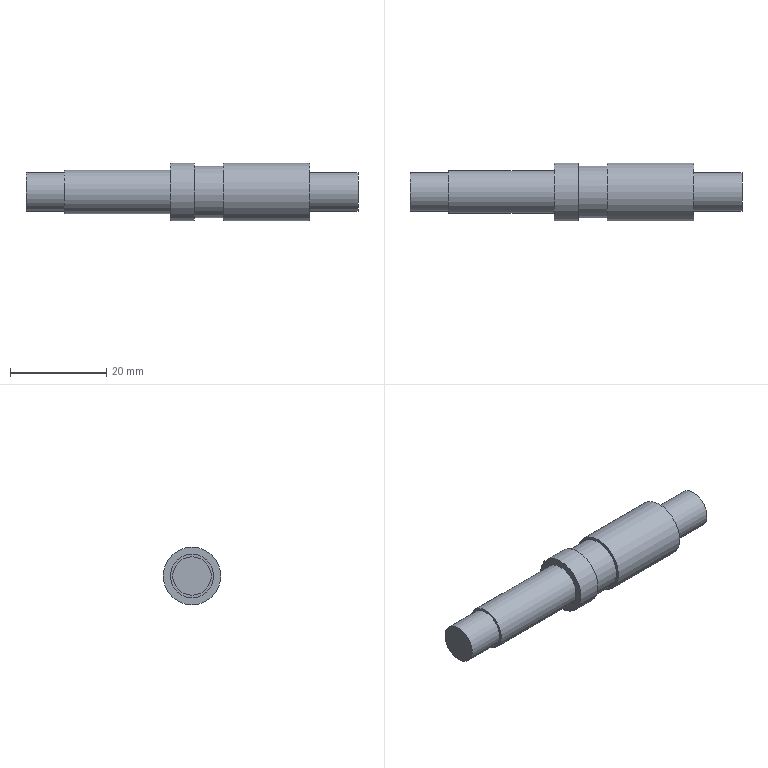Component | NX | VALVE_STEM | 1 solid | 13 faces | box 69 x 12 x 12 mm | volume 5453 mm3 | plane 7 | cylinder 6 | commonest cylinder face diameters 8 x2 12 x2 9 x1 10.782 x1
STEP:
#1=CARTESIAN_POINT('',(0.,0.,0.));
#2=DIRECTION('',(0.,0.,1.));
#3=DIRECTION('',(1.,0.,0.));
#4=AXIS2_PLACEMENT_3D('',#1,#2,#3);
#5=CARTESIAN_POINT('',(52.,-0.,16.));
#6=VERTEX_POINT('',#5);
#7=CARTESIAN_POINT('',(52.,-0.,20.));
#8=DIRECTION('',(1.,0.,0.));
#9=DIRECTION('',(0.,0.,-1.));
#10=AXIS2_PLACEMENT_3D('',#7,#8,#9);
#11=CIRCLE('',#10,4.);
#12=CARTESIAN_POINT('',(52.,-0.,20.));
#13=DIRECTION('',(-1.,0.,0.));
#14=DIRECTION('',(0.,0.,1.));
#15=AXIS2_PLACEMENT_3D('',#12,#13,#14);
#16=CYLINDRICAL_SURFACE('',#15,4.);
#17=CARTESIAN_POINT('',(9.425,0.));
#18=DIRECTION('',(-1.,0.));
#19=VECTOR('',#18,1.);
#20=LINE('',#17,#19);
#21=(GEOMETRIC_REPRESENTATION_CONTEXT(2)PARAMETRIC_REPRESENTATION_CONTEXT()REPRESENTATION_CONTEXT('',''));
#22=DEFINITIONAL_REPRESENTATION('',(#20),#21);
#23=PCURVE('',#16,#22);
#24=CARTESIAN_POINT('',(52.,-0.,20.));
#25=DIRECTION('',(1.,0.,0.));
#26=DIRECTION('',(0.,0.,-1.));
#27=AXIS2_PLACEMENT_3D('',#24,#25,#26);
#28=PLANE('',#27);
#29=CARTESIAN_POINT('',(0.,0.));
#30=DIRECTION('',(1.,0.));
#31=AXIS2_PLACEMENT_2D('',#29,#30);
#32=CIRCLE('',#31,4.);
#33=(GEOMETRIC_REPRESENTATION_CONTEXT(2)PARAMETRIC_REPRESENTATION_CONTEXT()REPRESENTATION_CONTEXT('',''));
#34=DEFINITIONAL_REPRESENTATION('',(#32),#33);
#35=PCURVE('',#28,#34);
#36=SURFACE_CURVE('',#11,(#23,#35),.PCURVE_S1.);
#37=EDGE_CURVE('',#6,#6,#36,.T.);
#38=ORIENTED_EDGE('',*,*,#37,.F.);
#39=CARTESIAN_POINT('',(44.,-0.,16.));
#40=VERTEX_POINT('',#39);
#41=CARTESIAN_POINT('',(52.,0.,16.));
#42=CARTESIAN_POINT('',(44.,0.,16.));
#43=B_SPLINE_CURVE_WITH_KNOTS('',1,(#41,#42),.UNSPECIFIED.,.F.,.F.,(2,2),(0.,8.),.PIECEWISE_BEZIER_KNOTS.);
#44=CARTESIAN_POINT('',(9.425,0.));
#45=DIRECTION('',(0.,1.));
#46=VECTOR('',#45,1.);
#47=LINE('',#44,#46);
#48=(GEOMETRIC_REPRESENTATION_CONTEXT(2)PARAMETRIC_REPRESENTATION_CONTEXT()REPRESENTATION_CONTEXT('',''));
#49=DEFINITIONAL_REPRESENTATION('',(#47),#48);
#50=PCURVE('',#16,#49);
#51=CARTESIAN_POINT('',(3.142,0.));
#52=DIRECTION('',(0.,1.));
#53=VECTOR('',#52,1.);
#54=LINE('',#51,#53);
#55=(GEOMETRIC_REPRESENTATION_CONTEXT(2)PARAMETRIC_REPRESENTATION_CONTEXT()REPRESENTATION_CONTEXT('',''));
#56=DEFINITIONAL_REPRESENTATION('',(#54),#55);
#57=PCURVE('',#16,#56);
#58=SEAM_CURVE('',#43,(#50,#57),.PCURVE_S1.);
#59=EDGE_CURVE('',#6,#40,#58,.T.);
#60=ORIENTED_EDGE('',*,*,#59,.T.);
#61=CARTESIAN_POINT('',(44.,-0.,20.));
#62=DIRECTION('',(1.,0.,0.));
#63=DIRECTION('',(0.,0.,-1.));
#64=AXIS2_PLACEMENT_3D('',#61,#62,#63);
#65=CIRCLE('',#64,4.);
#66=CARTESIAN_POINT('',(9.425,8.));
#67=DIRECTION('',(-1.,0.));
#68=VECTOR('',#67,1.);
#69=LINE('',#66,#68);
#70=(GEOMETRIC_REPRESENTATION_CONTEXT(2)PARAMETRIC_REPRESENTATION_CONTEXT()REPRESENTATION_CONTEXT('',''));
#71=DEFINITIONAL_REPRESENTATION('',(#69),#70);
#72=PCURVE('',#16,#71);
#73=CARTESIAN_POINT('',(44.,-0.,20.));
#74=DIRECTION('',(1.,0.,0.));
#75=DIRECTION('',(0.,0.,-1.));
#76=AXIS2_PLACEMENT_3D('',#73,#74,#75);
#77=PLANE('',#76);
#78=CARTESIAN_POINT('',(0.,0.));
#79=DIRECTION('',(1.,0.));
#80=AXIS2_PLACEMENT_2D('',#78,#79);
#81=CIRCLE('',#80,4.);
#82=(GEOMETRIC_REPRESENTATION_CONTEXT(2)PARAMETRIC_REPRESENTATION_CONTEXT()REPRESENTATION_CONTEXT('',''));
#83=DEFINITIONAL_REPRESENTATION('',(#81),#82);
#84=PCURVE('',#77,#83);
#85=SURFACE_CURVE('',#65,(#72,#84),.PCURVE_S1.);
#86=EDGE_CURVE('',#40,#40,#85,.T.);
#87=ORIENTED_EDGE('',*,*,#86,.T.);
#88=ORIENTED_EDGE('',*,*,#59,.F.);
#89=EDGE_LOOP('',(#38,#60,#87,#88));
#90=FACE_BOUND('',#89,.T.);
#91=ADVANCED_FACE('',(#90),#16,.T.);
#92=ORIENTED_EDGE('',*,*,#86,.F.);
#93=EDGE_LOOP('',(#92));
#94=FACE_BOUND('',#93,.T.);
#95=ADVANCED_FACE('',(#94),#77,.F.);
#96=CARTESIAN_POINT('',(52.,-0.,15.5));
#97=VERTEX_POINT('',#96);
#98=CARTESIAN_POINT('',(52.,-0.,20.));
#99=DIRECTION('',(1.,0.,0.));
#100=DIRECTION('',(0.,0.,-1.));
#101=AXIS2_PLACEMENT_3D('',#98,#99,#100);
#102=CIRCLE('',#101,4.5);
#103=CARTESIAN_POINT('',(74.,-0.,20.));
#104=DIRECTION('',(-1.,0.,0.));
#105=DIRECTION('',(0.,0.,1.));
#106=AXIS2_PLACEMENT_3D('',#103,#104,#105);
#107=CYLINDRICAL_SURFACE('',#106,4.5);
#108=CARTESIAN_POINT('',(9.425,22.));
#109=DIRECTION('',(-1.,0.));
#110=VECTOR('',#109,1.);
#111=LINE('',#108,#110);
#112=(GEOMETRIC_REPRESENTATION_CONTEXT(2)PARAMETRIC_REPRESENTATION_CONTEXT()REPRESENTATION_CONTEXT('',''));
#113=DEFINITIONAL_REPRESENTATION('',(#111),#112);
#114=PCURVE('',#107,#113);
#115=CARTESIAN_POINT('',(0.,0.));
#116=DIRECTION('',(1.,0.));
#117=AXIS2_PLACEMENT_2D('',#115,#116);
#118=CIRCLE('',#117,4.5);
#119=(GEOMETRIC_REPRESENTATION_CONTEXT(2)PARAMETRIC_REPRESENTATION_CONTEXT()REPRESENTATION_CONTEXT('',''));
#120=DEFINITIONAL_REPRESENTATION('',(#118),#119);
#121=PCURVE('',#28,#120);
#122=SURFACE_CURVE('',#102,(#114,#121),.PCURVE_S1.);
#123=EDGE_CURVE('',#97,#97,#122,.T.);
#124=ORIENTED_EDGE('',*,*,#123,.T.);
#125=CARTESIAN_POINT('',(74.,-0.,15.5));
#126=VERTEX_POINT('',#125);
#127=CARTESIAN_POINT('',(74.,0.,15.5));
#128=CARTESIAN_POINT('',(52.,0.,15.5));
#129=B_SPLINE_CURVE_WITH_KNOTS('',1,(#127,#128),.UNSPECIFIED.,.F.,.F.,(2,2),(0.,22.),.PIECEWISE_BEZIER_KNOTS.);
#130=CARTESIAN_POINT('',(3.142,0.));
#131=DIRECTION('',(0.,1.));
#132=VECTOR('',#131,1.);
#133=LINE('',#130,#132);
#134=(GEOMETRIC_REPRESENTATION_CONTEXT(2)PARAMETRIC_REPRESENTATION_CONTEXT()REPRESENTATION_CONTEXT('',''));
#135=DEFINITIONAL_REPRESENTATION('',(#133),#134);
#136=PCURVE('',#107,#135);
#137=CARTESIAN_POINT('',(9.425,0.));
#138=DIRECTION('',(0.,1.));
#139=VECTOR('',#138,1.);
#140=LINE('',#137,#139);
#141=(GEOMETRIC_REPRESENTATION_CONTEXT(2)PARAMETRIC_REPRESENTATION_CONTEXT()REPRESENTATION_CONTEXT('',''));
#142=DEFINITIONAL_REPRESENTATION('',(#140),#141);
#143=PCURVE('',#107,#142);
#144=SEAM_CURVE('',#129,(#136,#143),.PCURVE_S1.);
#145=EDGE_CURVE('',#126,#97,#144,.T.);
#146=ORIENTED_EDGE('',*,*,#145,.F.);
#147=CARTESIAN_POINT('',(74.,-0.,20.));
#148=DIRECTION('',(1.,0.,0.));
#149=DIRECTION('',(0.,0.,-1.));
#150=AXIS2_PLACEMENT_3D('',#147,#148,#149);
#151=CIRCLE('',#150,4.5);
#152=CARTESIAN_POINT('',(9.425,0.));
#153=DIRECTION('',(-1.,0.));
#154=VECTOR('',#153,1.);
#155=LINE('',#152,#154);
#156=(GEOMETRIC_REPRESENTATION_CONTEXT(2)PARAMETRIC_REPRESENTATION_CONTEXT()REPRESENTATION_CONTEXT('',''));
#157=DEFINITIONAL_REPRESENTATION('',(#155),#156);
#158=PCURVE('',#107,#157);
#159=CARTESIAN_POINT('',(74.,-0.,20.));
#160=DIRECTION('',(1.,0.,0.));
#161=DIRECTION('',(0.,0.,-1.));
#162=AXIS2_PLACEMENT_3D('',#159,#160,#161);
#163=PLANE('',#162);
#164=CARTESIAN_POINT('',(0.,0.));
#165=DIRECTION('',(1.,0.));
#166=AXIS2_PLACEMENT_2D('',#164,#165);
#167=CIRCLE('',#166,4.5);
#168=(GEOMETRIC_REPRESENTATION_CONTEXT(2)PARAMETRIC_REPRESENTATION_CONTEXT()REPRESENTATION_CONTEXT('',''));
#169=DEFINITIONAL_REPRESENTATION('',(#167),#168);
#170=PCURVE('',#163,#169);
#171=SURFACE_CURVE('',#151,(#158,#170),.PCURVE_S1.);
#172=EDGE_CURVE('',#126,#126,#171,.T.);
#173=ORIENTED_EDGE('',*,*,#172,.F.);
#174=ORIENTED_EDGE('',*,*,#145,.T.);
#175=EDGE_LOOP('',(#124,#146,#173,#174));
#176=FACE_BOUND('',#175,.T.);
#177=ADVANCED_FACE('',(#176),#107,.T.);
#178=ORIENTED_EDGE('',*,*,#37,.T.);
#179=EDGE_LOOP('',(#178));
#180=FACE_BOUND('',#179,.T.);
#181=ORIENTED_EDGE('',*,*,#123,.F.);
#182=EDGE_LOOP('',(#181));
#183=FACE_BOUND('',#182,.T.);
#184=ADVANCED_FACE('',(#180,#183),#28,.F.);
#185=CARTESIAN_POINT('',(79.,-0.,26.));
#186=VERTEX_POINT('',#185);
#187=CARTESIAN_POINT('',(79.,-0.,20.));
#188=DIRECTION('',(-1.,0.,0.));
#189=DIRECTION('',(0.,0.,1.));
#190=AXIS2_PLACEMENT_3D('',#187,#188,#189);
#191=CIRCLE('',#190,6.);
#192=CARTESIAN_POINT('',(103.,-0.,20.));
#193=DIRECTION('',(-1.,0.,0.));
#194=DIRECTION('',(0.,0.,1.));
#195=AXIS2_PLACEMENT_3D('',#192,#193,#194);
#196=CYLINDRICAL_SURFACE('',#195,6.);
#197=CARTESIAN_POINT('',(0.,24.));
#198=DIRECTION('',(1.,0.));
#199=VECTOR('',#198,1.);
#200=LINE('',#197,#199);
#201=(GEOMETRIC_REPRESENTATION_CONTEXT(2)PARAMETRIC_REPRESENTATION_CONTEXT()REPRESENTATION_CONTEXT('',''));
#202=DEFINITIONAL_REPRESENTATION('',(#200),#201);
#203=PCURVE('',#196,#202);
#204=CARTESIAN_POINT('',(79.,-0.,20.));
#205=DIRECTION('',(-1.,0.,0.));
#206=DIRECTION('',(0.,0.,1.));
#207=AXIS2_PLACEMENT_3D('',#204,#205,#206);
#208=PLANE('',#207);
#209=CARTESIAN_POINT('',(0.,0.));
#210=DIRECTION('',(1.,0.));
#211=AXIS2_PLACEMENT_2D('',#209,#210);
#212=CIRCLE('',#211,6.);
#213=(GEOMETRIC_REPRESENTATION_CONTEXT(2)PARAMETRIC_REPRESENTATION_CONTEXT()REPRESENTATION_CONTEXT('',''));
#214=DEFINITIONAL_REPRESENTATION('',(#212),#213);
#215=PCURVE('',#208,#214);
#216=SURFACE_CURVE('',#191,(#203,#215),.PCURVE_S1.);
#217=EDGE_CURVE('',#186,#186,#216,.T.);
#218=ORIENTED_EDGE('',*,*,#217,.T.);
#219=CARTESIAN_POINT('',(74.,-0.,26.));
#220=VERTEX_POINT('',#219);
#221=CARTESIAN_POINT('',(79.,-0.,26.));
#222=CARTESIAN_POINT('',(74.,-0.,26.));
#223=B_SPLINE_CURVE_WITH_KNOTS('',1,(#221,#222),.UNSPECIFIED.,.F.,.F.,(2,2),(24.,29.),.PIECEWISE_BEZIER_KNOTS.);
#224=CARTESIAN_POINT('',(6.283,0.));
#225=DIRECTION('',(0.,1.));
#226=VECTOR('',#225,1.);
#227=LINE('',#224,#226);
#228=(GEOMETRIC_REPRESENTATION_CONTEXT(2)PARAMETRIC_REPRESENTATION_CONTEXT()REPRESENTATION_CONTEXT('',''));
#229=DEFINITIONAL_REPRESENTATION('',(#227),#228);
#230=PCURVE('',#196,#229);
#231=CARTESIAN_POINT('',(0.,0.));
#232=DIRECTION('',(0.,1.));
#233=VECTOR('',#232,1.);
#234=LINE('',#231,#233);
#235=(GEOMETRIC_REPRESENTATION_CONTEXT(2)PARAMETRIC_REPRESENTATION_CONTEXT()REPRESENTATION_CONTEXT('',''));
#236=DEFINITIONAL_REPRESENTATION('',(#234),#235);
#237=PCURVE('',#196,#236);
#238=SEAM_CURVE('',#223,(#230,#237),.PCURVE_S1.);
#239=EDGE_CURVE('',#186,#220,#238,.T.);
#240=ORIENTED_EDGE('',*,*,#239,.T.);
#241=CARTESIAN_POINT('',(74.,-0.,14.));
#242=VERTEX_POINT('',#241);
#243=CARTESIAN_POINT('',(74.,-0.,20.));
#244=DIRECTION('',(1.,0.,0.));
#245=DIRECTION('',(0.,0.,-1.));
#246=AXIS2_PLACEMENT_3D('',#243,#244,#245);
#247=CIRCLE('',#246,6.);
#248=CARTESIAN_POINT('',(9.425,29.));
#249=DIRECTION('',(-1.,0.));
#250=VECTOR('',#249,1.);
#251=LINE('',#248,#250);
#252=(GEOMETRIC_REPRESENTATION_CONTEXT(2)PARAMETRIC_REPRESENTATION_CONTEXT()REPRESENTATION_CONTEXT('',''));
#253=DEFINITIONAL_REPRESENTATION('',(#251),#252);
#254=PCURVE('',#196,#253);
#255=CARTESIAN_POINT('',(0.,0.));
#256=DIRECTION('',(1.,0.));
#257=AXIS2_PLACEMENT_2D('',#255,#256);
#258=CIRCLE('',#257,6.);
#259=(GEOMETRIC_REPRESENTATION_CONTEXT(2)PARAMETRIC_REPRESENTATION_CONTEXT()REPRESENTATION_CONTEXT('',''));
#260=DEFINITIONAL_REPRESENTATION('',(#258),#259);
#261=PCURVE('',#163,#260);
#262=SURFACE_CURVE('',#247,(#254,#261),.PCURVE_S1.);
#263=EDGE_CURVE('',#220,#242,#262,.T.);
#264=ORIENTED_EDGE('',*,*,#263,.T.);
#265=CARTESIAN_POINT('',(74.,-0.,20.));
#266=DIRECTION('',(1.,0.,0.));
#267=DIRECTION('',(0.,0.,-1.));
#268=AXIS2_PLACEMENT_3D('',#265,#266,#267);
#269=CIRCLE('',#268,6.);
#270=CARTESIAN_POINT('',(3.142,29.));
#271=DIRECTION('',(-1.,0.));
#272=VECTOR('',#271,1.);
#273=LINE('',#270,#272);
#274=(GEOMETRIC_REPRESENTATION_CONTEXT(2)PARAMETRIC_REPRESENTATION_CONTEXT()REPRESENTATION_CONTEXT('',''));
#275=DEFINITIONAL_REPRESENTATION('',(#273),#274);
#276=PCURVE('',#196,#275);
#277=CARTESIAN_POINT('',(0.,0.));
#278=DIRECTION('',(1.,0.));
#279=AXIS2_PLACEMENT_2D('',#277,#278);
#280=CIRCLE('',#279,6.);
#281=(GEOMETRIC_REPRESENTATION_CONTEXT(2)PARAMETRIC_REPRESENTATION_CONTEXT()REPRESENTATION_CONTEXT('',''));
#282=DEFINITIONAL_REPRESENTATION('',(#280),#281);
#283=PCURVE('',#163,#282);
#284=SURFACE_CURVE('',#269,(#276,#283),.PCURVE_S1.);
#285=EDGE_CURVE('',#242,#220,#284,.T.);
#286=ORIENTED_EDGE('',*,*,#285,.T.);
#287=ORIENTED_EDGE('',*,*,#239,.F.);
#288=EDGE_LOOP('',(#218,#240,#264,#286,#287));
#289=FACE_BOUND('',#288,.T.);
#290=ADVANCED_FACE('',(#289),#196,.T.);
#291=ORIENTED_EDGE('',*,*,#172,.T.);
#292=EDGE_LOOP('',(#291));
#293=FACE_BOUND('',#292,.T.);
#294=ORIENTED_EDGE('',*,*,#285,.F.);
#295=ORIENTED_EDGE('',*,*,#263,.F.);
#296=EDGE_LOOP('',(#294,#295));
#297=FACE_BOUND('',#296,.T.);
#298=ADVANCED_FACE('',(#293,#297),#163,.F.);
#299=CARTESIAN_POINT('',(85.,-0.,14.609));
#300=VERTEX_POINT('',#299);
#301=CARTESIAN_POINT('',(85.,-0.,20.));
#302=DIRECTION('',(-1.,0.,0.));
#303=DIRECTION('',(0.,0.,-1.));
#304=AXIS2_PLACEMENT_3D('',#301,#302,#303);
#305=CIRCLE('',#304,5.391);
#306=CARTESIAN_POINT('',(85.,-0.,20.));
#307=DIRECTION('',(1.,0.,0.));
#308=DIRECTION('',(0.,0.,-1.));
#309=AXIS2_PLACEMENT_3D('',#306,#307,#308);
#310=PLANE('',#309);
#311=CARTESIAN_POINT('',(5.391,0.));
#312=CARTESIAN_POINT('',(5.391,-9.337));
#313=CARTESIAN_POINT('',(-2.696,-4.669));
#314=CARTESIAN_POINT('',(-10.782,-0.));
#315=CARTESIAN_POINT('',(-2.696,4.669));
#316=CARTESIAN_POINT('',(5.391,9.337));
#317=CARTESIAN_POINT('',(5.391,0.));
#318=(BOUNDED_CURVE()B_SPLINE_CURVE(2,(#311,#312,#313,#314,#315,#316,#317),.UNSPECIFIED.,.T.,.F.)B_SPLINE_CURVE_WITH_KNOTS((1,2,2,2,2,1),(-2.094,0.,2.094,4.189,6.283,8.378),.UNSPECIFIED.)CURVE()GEOMETRIC_REPRESENTATION_ITEM()RATIONAL_B_SPLINE_CURVE((1.,0.5,1.,0.5,1.,0.5,1.))REPRESENTATION_ITEM(''));
#319=(GEOMETRIC_REPRESENTATION_CONTEXT(2)PARAMETRIC_REPRESENTATION_CONTEXT()REPRESENTATION_CONTEXT('',''));
#320=DEFINITIONAL_REPRESENTATION('',(#318),#319);
#321=PCURVE('',#310,#320);
#322=CARTESIAN_POINT('',(78.,-0.,20.));
#323=DIRECTION('',(1.,0.,0.));
#324=DIRECTION('',(0.,0.,-1.));
#325=AXIS2_PLACEMENT_3D('',#322,#323,#324);
#326=CYLINDRICAL_SURFACE('',#325,5.391);
#327=CARTESIAN_POINT('',(6.283,7.));
#328=DIRECTION('',(-1.,0.));
#329=VECTOR('',#328,1.);
#330=LINE('',#327,#329);
#331=(GEOMETRIC_REPRESENTATION_CONTEXT(2)PARAMETRIC_REPRESENTATION_CONTEXT()REPRESENTATION_CONTEXT('',''));
#332=DEFINITIONAL_REPRESENTATION('',(#330),#331);
#333=PCURVE('',#326,#332);
#334=SURFACE_CURVE('',#305,(#321,#333),.PCURVE_S1.);
#335=EDGE_CURVE('',#300,#300,#334,.T.);
#336=ORIENTED_EDGE('',*,*,#335,.F.);
#337=EDGE_LOOP('',(#336));
#338=FACE_BOUND('',#337,.T.);
#339=CARTESIAN_POINT('',(85.,-0.,14.));
#340=VERTEX_POINT('',#339);
#341=CARTESIAN_POINT('',(85.,-0.,20.));
#342=DIRECTION('',(1.,0.,0.));
#343=DIRECTION('',(0.,0.,-1.));
#344=AXIS2_PLACEMENT_3D('',#341,#342,#343);
#345=CIRCLE('',#344,6.);
#346=CARTESIAN_POINT('',(0.,0.));
#347=DIRECTION('',(1.,0.));
#348=AXIS2_PLACEMENT_2D('',#346,#347);
#349=CIRCLE('',#348,6.);
#350=(GEOMETRIC_REPRESENTATION_CONTEXT(2)PARAMETRIC_REPRESENTATION_CONTEXT()REPRESENTATION_CONTEXT('',''));
#351=DEFINITIONAL_REPRESENTATION('',(#349),#350);
#352=PCURVE('',#310,#351);
#353=CARTESIAN_POINT('',(103.,-0.,20.));
#354=DIRECTION('',(-1.,0.,0.));
#355=DIRECTION('',(0.,0.,1.));
#356=AXIS2_PLACEMENT_3D('',#353,#354,#355);
#357=CYLINDRICAL_SURFACE('',#356,6.);
#358=CARTESIAN_POINT('',(9.425,18.));
#359=DIRECTION('',(-1.,0.));
#360=VECTOR('',#359,1.);
#361=LINE('',#358,#360);
#362=(GEOMETRIC_REPRESENTATION_CONTEXT(2)PARAMETRIC_REPRESENTATION_CONTEXT()REPRESENTATION_CONTEXT('',''));
#363=DEFINITIONAL_REPRESENTATION('',(#361),#362);
#364=PCURVE('',#357,#363);
#365=SURFACE_CURVE('',#345,(#352,#364),.PCURVE_S1.);
#366=EDGE_CURVE('',#340,#340,#365,.T.);
#367=ORIENTED_EDGE('',*,*,#366,.F.);
#368=EDGE_LOOP('',(#367));
#369=FACE_BOUND('',#368,.T.);
#370=ADVANCED_FACE('',(#338,#369),#310,.F.);
#371=CARTESIAN_POINT('',(79.,-0.,25.391));
#372=VERTEX_POINT('',#371);
#373=CARTESIAN_POINT('',(79.,-0.,14.609));
#374=VERTEX_POINT('',#373);
#375=CARTESIAN_POINT('',(79.,-0.,20.));
#376=DIRECTION('',(1.,0.,0.));
#377=DIRECTION('',(0.,0.,1.));
#378=AXIS2_PLACEMENT_3D('',#375,#376,#377);
#379=CIRCLE('',#378,5.391);
#380=CARTESIAN_POINT('',(5.391,0.));
#381=CARTESIAN_POINT('',(5.391,-9.337));
#382=CARTESIAN_POINT('',(-2.696,-4.669));
#383=CARTESIAN_POINT('',(-10.782,-0.));
#384=CARTESIAN_POINT('',(-2.696,4.669));
#385=CARTESIAN_POINT('',(5.391,9.337));
#386=CARTESIAN_POINT('',(5.391,0.));
#387=(BOUNDED_CURVE()B_SPLINE_CURVE(2,(#380,#381,#382,#383,#384,#385,#386),.UNSPECIFIED.,.T.,.F.)B_SPLINE_CURVE_WITH_KNOTS((1,2,2,2,2,1),(-2.094,0.,2.094,4.189,6.283,8.378),.UNSPECIFIED.)CURVE()GEOMETRIC_REPRESENTATION_ITEM()RATIONAL_B_SPLINE_CURVE((1.,0.5,1.,0.5,1.,0.5,1.))REPRESENTATION_ITEM(''));
#388=(GEOMETRIC_REPRESENTATION_CONTEXT(2)PARAMETRIC_REPRESENTATION_CONTEXT()REPRESENTATION_CONTEXT('',''));
#389=DEFINITIONAL_REPRESENTATION('',(#387),#388);
#390=PCURVE('',#208,#389);
#391=CARTESIAN_POINT('',(3.142,1.));
#392=DIRECTION('',(1.,0.));
#393=VECTOR('',#392,1.);
#394=LINE('',#391,#393);
#395=(GEOMETRIC_REPRESENTATION_CONTEXT(2)PARAMETRIC_REPRESENTATION_CONTEXT()REPRESENTATION_CONTEXT('',''));
#396=DEFINITIONAL_REPRESENTATION('',(#394),#395);
#397=PCURVE('',#326,#396);
#398=SURFACE_CURVE('',#379,(#390,#397),.PCURVE_S1.);
#399=EDGE_CURVE('',#372,#374,#398,.T.);
#400=ORIENTED_EDGE('',*,*,#399,.F.);
#401=CARTESIAN_POINT('',(79.,-0.,20.));
#402=DIRECTION('',(1.,0.,0.));
#403=DIRECTION('',(0.,0.,1.));
#404=AXIS2_PLACEMENT_3D('',#401,#402,#403);
#405=CIRCLE('',#404,5.391);
#406=CARTESIAN_POINT('',(5.391,0.));
#407=CARTESIAN_POINT('',(5.391,-9.337));
#408=CARTESIAN_POINT('',(-2.696,-4.669));
#409=CARTESIAN_POINT('',(-10.782,-0.));
#410=CARTESIAN_POINT('',(-2.696,4.669));
#411=CARTESIAN_POINT('',(5.391,9.337));
#412=CARTESIAN_POINT('',(5.391,0.));
#413=(BOUNDED_CURVE()B_SPLINE_CURVE(2,(#406,#407,#408,#409,#410,#411,#412),.UNSPECIFIED.,.T.,.F.)B_SPLINE_CURVE_WITH_KNOTS((1,2,2,2,2,1),(-2.094,0.,2.094,4.189,6.283,8.378),.UNSPECIFIED.)CURVE()GEOMETRIC_REPRESENTATION_ITEM()RATIONAL_B_SPLINE_CURVE((1.,0.5,1.,0.5,1.,0.5,1.))REPRESENTATION_ITEM(''));
#414=(GEOMETRIC_REPRESENTATION_CONTEXT(2)PARAMETRIC_REPRESENTATION_CONTEXT()REPRESENTATION_CONTEXT('',''));
#415=DEFINITIONAL_REPRESENTATION('',(#413),#414);
#416=PCURVE('',#208,#415);
#417=CARTESIAN_POINT('',(-3.142,1.));
#418=DIRECTION('',(1.,0.));
#419=VECTOR('',#418,1.);
#420=LINE('',#417,#419);
#421=(GEOMETRIC_REPRESENTATION_CONTEXT(2)PARAMETRIC_REPRESENTATION_CONTEXT()REPRESENTATION_CONTEXT('',''));
#422=DEFINITIONAL_REPRESENTATION('',(#420),#421);
#423=PCURVE('',#326,#422);
#424=SURFACE_CURVE('',#405,(#416,#423),.PCURVE_S1.);
#425=EDGE_CURVE('',#374,#372,#424,.T.);
#426=ORIENTED_EDGE('',*,*,#425,.F.);
#427=EDGE_LOOP('',(#400,#426));
#428=FACE_BOUND('',#427,.T.);
#429=ORIENTED_EDGE('',*,*,#217,.F.);
#430=EDGE_LOOP('',(#429));
#431=FACE_BOUND('',#430,.T.);
#432=ADVANCED_FACE('',(#428,#431),#208,.F.);
#433=ORIENTED_EDGE('',*,*,#335,.T.);
#434=CARTESIAN_POINT('',(79.,-0.,14.609));
#435=CARTESIAN_POINT('',(85.,-0.,14.609));
#436=B_SPLINE_CURVE_WITH_KNOTS('',1,(#434,#435),.UNSPECIFIED.,.F.,.F.,(2,2),(1.,7.),.PIECEWISE_BEZIER_KNOTS.);
#437=CARTESIAN_POINT('',(0.,0.));
#438=DIRECTION('',(0.,1.));
#439=VECTOR('',#438,1.);
#440=LINE('',#437,#439);
#441=(GEOMETRIC_REPRESENTATION_CONTEXT(2)PARAMETRIC_REPRESENTATION_CONTEXT()REPRESENTATION_CONTEXT('',''));
#442=DEFINITIONAL_REPRESENTATION('',(#440),#441);
#443=PCURVE('',#326,#442);
#444=CARTESIAN_POINT('',(6.283,0.));
#445=DIRECTION('',(0.,1.));
#446=VECTOR('',#445,1.);
#447=LINE('',#444,#446);
#448=(GEOMETRIC_REPRESENTATION_CONTEXT(2)PARAMETRIC_REPRESENTATION_CONTEXT()REPRESENTATION_CONTEXT('',''));
#449=DEFINITIONAL_REPRESENTATION('',(#447),#448);
#450=PCURVE('',#326,#449);
#451=SEAM_CURVE('',#436,(#443,#450),.PCURVE_S1.);
#452=EDGE_CURVE('',#374,#300,#451,.T.);
#453=ORIENTED_EDGE('',*,*,#452,.F.);
#454=ORIENTED_EDGE('',*,*,#425,.T.);
#455=ORIENTED_EDGE('',*,*,#399,.T.);
#456=ORIENTED_EDGE('',*,*,#452,.T.);
#457=EDGE_LOOP('',(#433,#453,#454,#455,#456));
#458=FACE_BOUND('',#457,.T.);
#459=ADVANCED_FACE('',(#458),#326,.T.);
#460=CARTESIAN_POINT('',(113.,-0.,16.));
#461=VERTEX_POINT('',#460);
#462=CARTESIAN_POINT('',(113.,-0.,20.));
#463=DIRECTION('',(1.,0.,0.));
#464=DIRECTION('',(0.,0.,-1.));
#465=AXIS2_PLACEMENT_3D('',#462,#463,#464);
#466=CIRCLE('',#465,4.);
#467=CARTESIAN_POINT('',(113.,-0.,20.));
#468=DIRECTION('',(1.,0.,0.));
#469=DIRECTION('',(0.,0.,-1.));
#470=AXIS2_PLACEMENT_3D('',#467,#468,#469);
#471=PLANE('',#470);
#472=CARTESIAN_POINT('',(0.,0.));
#473=DIRECTION('',(1.,0.));
#474=AXIS2_PLACEMENT_2D('',#472,#473);
#475=CIRCLE('',#474,4.);
#476=(GEOMETRIC_REPRESENTATION_CONTEXT(2)PARAMETRIC_REPRESENTATION_CONTEXT()REPRESENTATION_CONTEXT('',''));
#477=DEFINITIONAL_REPRESENTATION('',(#475),#476);
#478=PCURVE('',#471,#477);
#479=CARTESIAN_POINT('',(113.,-0.,20.));
#480=DIRECTION('',(-1.,0.,0.));
#481=DIRECTION('',(0.,0.,1.));
#482=AXIS2_PLACEMENT_3D('',#479,#480,#481);
#483=CYLINDRICAL_SURFACE('',#482,4.);
#484=CARTESIAN_POINT('',(9.425,0.));
#485=DIRECTION('',(-1.,0.));
#486=VECTOR('',#485,1.);
#487=LINE('',#484,#486);
#488=(GEOMETRIC_REPRESENTATION_CONTEXT(2)PARAMETRIC_REPRESENTATION_CONTEXT()REPRESENTATION_CONTEXT('',''));
#489=DEFINITIONAL_REPRESENTATION('',(#487),#488);
#490=PCURVE('',#483,#489);
#491=SURFACE_CURVE('',#466,(#478,#490),.PCURVE_S1.);
#492=EDGE_CURVE('',#461,#461,#491,.T.);
#493=ORIENTED_EDGE('',*,*,#492,.T.);
#494=EDGE_LOOP('',(#493));
#495=FACE_BOUND('',#494,.T.);
#496=ADVANCED_FACE('',(#495),#471,.T.);
#497=ORIENTED_EDGE('',*,*,#492,.F.);
#498=CARTESIAN_POINT('',(103.,-0.,16.));
#499=VERTEX_POINT('',#498);
#500=CARTESIAN_POINT('',(113.,0.,16.));
#501=CARTESIAN_POINT('',(103.,0.,16.));
#502=B_SPLINE_CURVE_WITH_KNOTS('',1,(#500,#501),.UNSPECIFIED.,.F.,.F.,(2,2),(0.,10.),.PIECEWISE_BEZIER_KNOTS.);
#503=CARTESIAN_POINT('',(9.425,0.));
#504=DIRECTION('',(0.,1.));
#505=VECTOR('',#504,1.);
#506=LINE('',#503,#505);
#507=(GEOMETRIC_REPRESENTATION_CONTEXT(2)PARAMETRIC_REPRESENTATION_CONTEXT()REPRESENTATION_CONTEXT('',''));
#508=DEFINITIONAL_REPRESENTATION('',(#506),#507);
#509=PCURVE('',#483,#508);
#510=CARTESIAN_POINT('',(3.142,0.));
#511=DIRECTION('',(0.,1.));
#512=VECTOR('',#511,1.);
#513=LINE('',#510,#512);
#514=(GEOMETRIC_REPRESENTATION_CONTEXT(2)PARAMETRIC_REPRESENTATION_CONTEXT()REPRESENTATION_CONTEXT('',''));
#515=DEFINITIONAL_REPRESENTATION('',(#513),#514);
#516=PCURVE('',#483,#515);
#517=SEAM_CURVE('',#502,(#509,#516),.PCURVE_S1.);
#518=EDGE_CURVE('',#461,#499,#517,.T.);
#519=ORIENTED_EDGE('',*,*,#518,.T.);
#520=CARTESIAN_POINT('',(103.,-0.,20.));
#521=DIRECTION('',(1.,0.,0.));
#522=DIRECTION('',(0.,0.,-1.));
#523=AXIS2_PLACEMENT_3D('',#520,#521,#522);
#524=CIRCLE('',#523,4.);
#525=CARTESIAN_POINT('',(9.425,10.));
#526=DIRECTION('',(-1.,0.));
#527=VECTOR('',#526,1.);
#528=LINE('',#525,#527);
#529=(GEOMETRIC_REPRESENTATION_CONTEXT(2)PARAMETRIC_REPRESENTATION_CONTEXT()REPRESENTATION_CONTEXT('',''));
#530=DEFINITIONAL_REPRESENTATION('',(#528),#529);
#531=PCURVE('',#483,#530);
#532=CARTESIAN_POINT('',(103.,-0.,20.));
#533=DIRECTION('',(1.,0.,0.));
#534=DIRECTION('',(0.,0.,-1.));
#535=AXIS2_PLACEMENT_3D('',#532,#533,#534);
#536=PLANE('',#535);
#537=CARTESIAN_POINT('',(0.,0.));
#538=DIRECTION('',(1.,0.));
#539=AXIS2_PLACEMENT_2D('',#537,#538);
#540=CIRCLE('',#539,4.);
#541=(GEOMETRIC_REPRESENTATION_CONTEXT(2)PARAMETRIC_REPRESENTATION_CONTEXT()REPRESENTATION_CONTEXT('',''));
#542=DEFINITIONAL_REPRESENTATION('',(#540),#541);
#543=PCURVE('',#536,#542);
#544=SURFACE_CURVE('',#524,(#531,#543),.PCURVE_S1.);
#545=EDGE_CURVE('',#499,#499,#544,.T.);
#546=ORIENTED_EDGE('',*,*,#545,.T.);
#547=ORIENTED_EDGE('',*,*,#518,.F.);
#548=EDGE_LOOP('',(#497,#519,#546,#547));
#549=FACE_BOUND('',#548,.T.);
#550=ADVANCED_FACE('',(#549),#483,.T.);
#551=ORIENTED_EDGE('',*,*,#545,.F.);
#552=EDGE_LOOP('',(#551));
#553=FACE_BOUND('',#552,.T.);
#554=CARTESIAN_POINT('',(103.,-0.,14.));
#555=VERTEX_POINT('',#554);
#556=CARTESIAN_POINT('',(103.,-0.,20.));
#557=DIRECTION('',(1.,0.,0.));
#558=DIRECTION('',(0.,0.,-1.));
#559=AXIS2_PLACEMENT_3D('',#556,#557,#558);
#560=CIRCLE('',#559,6.);
#561=CARTESIAN_POINT('',(0.,0.));
#562=DIRECTION('',(1.,0.));
#563=AXIS2_PLACEMENT_2D('',#561,#562);
#564=CIRCLE('',#563,6.);
#565=(GEOMETRIC_REPRESENTATION_CONTEXT(2)PARAMETRIC_REPRESENTATION_CONTEXT()REPRESENTATION_CONTEXT('',''));
#566=DEFINITIONAL_REPRESENTATION('',(#564),#565);
#567=PCURVE('',#536,#566);
#568=CARTESIAN_POINT('',(9.425,0.));
#569=DIRECTION('',(-1.,0.));
#570=VECTOR('',#569,1.);
#571=LINE('',#568,#570);
#572=(GEOMETRIC_REPRESENTATION_CONTEXT(2)PARAMETRIC_REPRESENTATION_CONTEXT()REPRESENTATION_CONTEXT('',''));
#573=DEFINITIONAL_REPRESENTATION('',(#571),#572);
#574=PCURVE('',#357,#573);
#575=SURFACE_CURVE('',#560,(#567,#574),.PCURVE_S1.);
#576=EDGE_CURVE('',#555,#555,#575,.T.);
#577=ORIENTED_EDGE('',*,*,#576,.T.);
#578=EDGE_LOOP('',(#577));
#579=FACE_BOUND('',#578,.T.);
#580=ADVANCED_FACE('',(#553,#579),#536,.T.);
#581=ORIENTED_EDGE('',*,*,#366,.T.);
#582=CARTESIAN_POINT('',(103.,0.,14.));
#583=CARTESIAN_POINT('',(85.,0.,14.));
#584=B_SPLINE_CURVE_WITH_KNOTS('',1,(#582,#583),.UNSPECIFIED.,.F.,.F.,(2,2),(0.,18.),.PIECEWISE_BEZIER_KNOTS.);
#585=CARTESIAN_POINT('',(3.142,0.));
#586=DIRECTION('',(0.,1.));
#587=VECTOR('',#586,1.);
#588=LINE('',#585,#587);
#589=(GEOMETRIC_REPRESENTATION_CONTEXT(2)PARAMETRIC_REPRESENTATION_CONTEXT()REPRESENTATION_CONTEXT('',''));
#590=DEFINITIONAL_REPRESENTATION('',(#588),#589);
#591=PCURVE('',#357,#590);
#592=CARTESIAN_POINT('',(9.425,0.));
#593=DIRECTION('',(0.,1.));
#594=VECTOR('',#593,1.);
#595=LINE('',#592,#594);
#596=(GEOMETRIC_REPRESENTATION_CONTEXT(2)PARAMETRIC_REPRESENTATION_CONTEXT()REPRESENTATION_CONTEXT('',''));
#597=DEFINITIONAL_REPRESENTATION('',(#595),#596);
#598=PCURVE('',#357,#597);
#599=SEAM_CURVE('',#584,(#591,#598),.PCURVE_S1.);
#600=EDGE_CURVE('',#555,#340,#599,.T.);
#601=ORIENTED_EDGE('',*,*,#600,.F.);
#602=ORIENTED_EDGE('',*,*,#576,.F.);
#603=ORIENTED_EDGE('',*,*,#600,.T.);
#604=EDGE_LOOP('',(#581,#601,#602,#603));
#605=FACE_BOUND('',#604,.T.);
#606=ADVANCED_FACE('',(#605),#357,.T.);
#607=CLOSED_SHELL('',(#91,#95,#177,#184,#290,#298,#370,#432,#459,#496,#550,#580,#606));
#608=MANIFOLD_SOLID_BREP('',#607);
#609=(LENGTH_UNIT()NAMED_UNIT(*)SI_UNIT(.MILLI.,.METRE.));
#610=UNCERTAINTY_MEASURE_WITH_UNIT(LENGTH_MEASURE(0.000005),#609,'','');
#611=(NAMED_UNIT(*)PLANE_ANGLE_UNIT()SI_UNIT($,.RADIAN.));
#612=(NAMED_UNIT(*)SI_UNIT($,.STERADIAN.)SOLID_ANGLE_UNIT());
#613=(GEOMETRIC_REPRESENTATION_CONTEXT(3)GLOBAL_UNCERTAINTY_ASSIGNED_CONTEXT((#610))GLOBAL_UNIT_ASSIGNED_CONTEXT((#609,#611,#612))REPRESENTATION_CONTEXT('',''));
#614=ADVANCED_BREP_SHAPE_REPRESENTATION('',(#4,#608),#613);